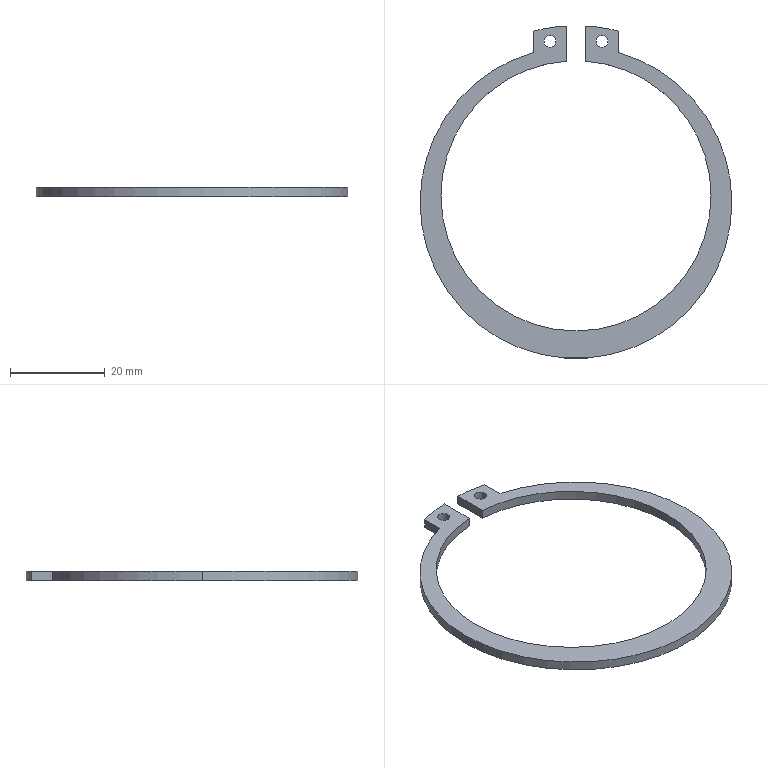Component | SolidWorks | shaft circlip GB894-1 d60-1 | 1 solid | 18 faces | box 65.8 x 70.14 x 2 mm | volume 1778 mm3 | cylinder 12 | plane 6 | commonest cylinder face diameters 2.5 x4 65.8 x3 57 x3 71.8 x2
build123d program:
from build123d import *

# Parameters (mm, degrees)
RING_PROFILE_GB894_1_60_INSTALLED_R = 1.25
RING_BODY_S2_DEPTH                  = 2


with BuildPart() as part:
    # Ring profile GB894.1-60 installed → Ring body s2 (new body)
    with BuildSketch(Plane.XY):
        with BuildLine():
            Line((2, 28.43), (2, 35.844))
            ThreePointArc((2, 35.844), (5.527, 35.472), (9, 34.754))
            Line((9, 34.754), (9, 30.245))
            ThreePointArc((9, 30.245), (0, -34.3), (-9, 30.245))
            Line((-9, 30.245), (-9, 34.754))
            ThreePointArc((-9, 34.754), (-5.527, 35.472), (-2, 35.844))
            Line((-2, 35.844), (-2, 28.43))
            ThreePointArc((-2, 28.43), (0, -28.5), (2, 28.43))
        make_face()
        with Locations((5.5, 32.6)):
            Circle(RING_PROFILE_GB894_1_60_INSTALLED_R, mode=Mode.SUBTRACT)
        with Locations((-5.5, 32.6)):
            Circle(RING_PROFILE_GB894_1_60_INSTALLED_R, mode=Mode.SUBTRACT)
    extrude(amount=RING_BODY_S2_DEPTH)


solid = part.part

# Placed as in the assembly
solid = solid.moved(Location((-85, 178, 139), (0, 0, 0)))
STEP:
#1=CARTESIAN_POINT('',(-3.612,8.291,5.551));
#2=VERTEX_POINT('',#1);
#3=CARTESIAN_POINT('',(-3.514,8.291,5.551));
#4=VERTEX_POINT('',#3);
#5=CARTESIAN_POINT('',(-3.563,8.291,5.551));
#6=DIRECTION('',(0.,0.,1.));
#7=DIRECTION('',(1.,0.,0.));
#8=AXIS2_PLACEMENT_3D('',#5,#6,#7);
#9=CIRCLE('',#8,0.04921);
#10=EDGE_CURVE('',#2,#4,#9,.T.);
#11=ORIENTED_EDGE('',*,*,#10,.T.);
#12=CARTESIAN_POINT('',(-3.514,8.291,5.472));
#13=VERTEX_POINT('',#12);
#14=CARTESIAN_POINT('',(-3.514,8.291,5.551));
#15=DIRECTION('',(0.,0.,-1.));
#16=VECTOR('',#15,39.37);
#17=LINE('',#14,#16);
#18=EDGE_CURVE('',#4,#13,#17,.T.);
#19=ORIENTED_EDGE('',*,*,#18,.T.);
#20=CARTESIAN_POINT('',(-3.612,8.291,5.472));
#21=VERTEX_POINT('',#20);
#22=CARTESIAN_POINT('',(-3.563,8.291,5.472));
#23=DIRECTION('',(0.,0.,1.));
#24=DIRECTION('',(1.,0.,0.));
#25=AXIS2_PLACEMENT_3D('',#22,#23,#24);
#26=CIRCLE('',#25,0.04921);
#27=EDGE_CURVE('',#21,#13,#26,.T.);
#28=ORIENTED_EDGE('',*,*,#27,.F.);
#29=CARTESIAN_POINT('',(-3.612,8.291,5.551));
#30=DIRECTION('',(0.,0.,-1.));
#31=VECTOR('',#30,39.37);
#32=LINE('',#29,#31);
#33=EDGE_CURVE('',#2,#21,#32,.T.);
#34=ORIENTED_EDGE('',*,*,#33,.F.);
#35=EDGE_LOOP('',(#11,#19,#28,#34));
#36=FACE_OUTER_BOUND('',#35,.T.);
#37=CARTESIAN_POINT('',(-3.563,8.291,5.551));
#38=DIRECTION('',(0.,0.,-1.));
#39=DIRECTION('',(-1.,0.,0.));
#40=AXIS2_PLACEMENT_3D('',#37,#38,#39);
#41=CYLINDRICAL_SURFACE('',#40,0.04921);
#42=ADVANCED_FACE('',(#36),#41,.F.);
#43=CARTESIAN_POINT('',(-3.179,8.291,5.551));
#44=VERTEX_POINT('',#43);
#45=CARTESIAN_POINT('',(-3.081,8.291,5.551));
#46=VERTEX_POINT('',#45);
#47=CARTESIAN_POINT('',(-3.13,8.291,5.551));
#48=DIRECTION('',(0.,0.,1.));
#49=DIRECTION('',(1.,0.,0.));
#50=AXIS2_PLACEMENT_3D('',#47,#48,#49);
#51=CIRCLE('',#50,0.04921);
#52=EDGE_CURVE('',#44,#46,#51,.T.);
#53=ORIENTED_EDGE('',*,*,#52,.T.);
#54=CARTESIAN_POINT('',(-3.081,8.291,5.472));
#55=VERTEX_POINT('',#54);
#56=CARTESIAN_POINT('',(-3.081,8.291,5.551));
#57=DIRECTION('',(0.,0.,-1.));
#58=VECTOR('',#57,39.37);
#59=LINE('',#56,#58);
#60=EDGE_CURVE('',#46,#55,#59,.T.);
#61=ORIENTED_EDGE('',*,*,#60,.T.);
#62=CARTESIAN_POINT('',(-3.179,8.291,5.472));
#63=VERTEX_POINT('',#62);
#64=CARTESIAN_POINT('',(-3.13,8.291,5.472));
#65=DIRECTION('',(0.,0.,1.));
#66=DIRECTION('',(1.,0.,0.));
#67=AXIS2_PLACEMENT_3D('',#64,#65,#66);
#68=CIRCLE('',#67,0.04921);
#69=EDGE_CURVE('',#63,#55,#68,.T.);
#70=ORIENTED_EDGE('',*,*,#69,.F.);
#71=CARTESIAN_POINT('',(-3.179,8.291,5.551));
#72=DIRECTION('',(0.,0.,-1.));
#73=VECTOR('',#72,39.37);
#74=LINE('',#71,#73);
#75=EDGE_CURVE('',#44,#63,#74,.T.);
#76=ORIENTED_EDGE('',*,*,#75,.F.);
#77=EDGE_LOOP('',(#53,#61,#70,#76));
#78=FACE_OUTER_BOUND('',#77,.T.);
#79=CARTESIAN_POINT('',(-3.13,8.291,5.551));
#80=DIRECTION('',(0.,0.,-1.));
#81=DIRECTION('',(-1.,0.,0.));
#82=AXIS2_PLACEMENT_3D('',#79,#80,#81);
#83=CYLINDRICAL_SURFACE('',#82,0.04921);
#84=ADVANCED_FACE('',(#78),#83,.F.);
#85=CARTESIAN_POINT('',(-2.051,6.953,5.551));
#86=VERTEX_POINT('',#85);
#87=CARTESIAN_POINT('',(-2.992,8.199,5.551));
#88=VERTEX_POINT('',#87);
#89=CARTESIAN_POINT('',(-3.346,6.953,5.551));
#90=DIRECTION('',(0.,0.,1.));
#91=DIRECTION('',(-1.,0.,0.));
#92=AXIS2_PLACEMENT_3D('',#89,#90,#91);
#93=CIRCLE('',#92,1.295);
#94=EDGE_CURVE('',#86,#88,#93,.T.);
#95=ORIENTED_EDGE('',*,*,#94,.F.);
#96=CARTESIAN_POINT('',(-2.051,6.953,5.472));
#97=VERTEX_POINT('',#96);
#98=CARTESIAN_POINT('',(-2.051,6.953,5.551));
#99=DIRECTION('',(0.,0.,-1.));
#100=VECTOR('',#99,39.37);
#101=LINE('',#98,#100);
#102=EDGE_CURVE('',#86,#97,#101,.T.);
#103=ORIENTED_EDGE('',*,*,#102,.T.);
#104=CARTESIAN_POINT('',(-2.992,8.199,5.472));
#105=VERTEX_POINT('',#104);
#106=CARTESIAN_POINT('',(-3.346,6.953,5.472));
#107=DIRECTION('',(0.,0.,1.));
#108=DIRECTION('',(-1.,0.,0.));
#109=AXIS2_PLACEMENT_3D('',#106,#107,#108);
#110=CIRCLE('',#109,1.295);
#111=EDGE_CURVE('',#97,#105,#110,.T.);
#112=ORIENTED_EDGE('',*,*,#111,.T.);
#113=CARTESIAN_POINT('',(-2.992,8.199,5.551));
#114=DIRECTION('',(0.,0.,-1.));
#115=VECTOR('',#114,39.37);
#116=LINE('',#113,#115);
#117=EDGE_CURVE('',#88,#105,#116,.T.);
#118=ORIENTED_EDGE('',*,*,#117,.F.);
#119=EDGE_LOOP('',(#95,#103,#112,#118));
#120=FACE_OUTER_BOUND('',#119,.T.);
#121=CARTESIAN_POINT('',(-3.346,6.953,5.551));
#122=DIRECTION('',(0.,0.,-1.));
#123=DIRECTION('',(-1.,0.,0.));
#124=AXIS2_PLACEMENT_3D('',#121,#122,#123);
#125=CYLINDRICAL_SURFACE('',#124,1.295);
#126=ADVANCED_FACE('',(#120),#125,.T.);
#127=ORIENTED_EDGE('',*,*,#102,.F.);
#128=CARTESIAN_POINT('',(-4.642,6.953,5.551));
#129=VERTEX_POINT('',#128);
#130=CARTESIAN_POINT('',(-3.346,6.953,5.551));
#131=DIRECTION('',(0.,0.,1.));
#132=DIRECTION('',(-1.,0.,0.));
#133=AXIS2_PLACEMENT_3D('',#130,#131,#132);
#134=CIRCLE('',#133,1.295);
#135=EDGE_CURVE('',#129,#86,#134,.T.);
#136=ORIENTED_EDGE('',*,*,#135,.F.);
#137=CARTESIAN_POINT('',(-4.642,6.953,5.472));
#138=VERTEX_POINT('',#137);
#139=CARTESIAN_POINT('',(-4.642,6.953,5.551));
#140=DIRECTION('',(0.,0.,-1.));
#141=VECTOR('',#140,39.37);
#142=LINE('',#139,#141);
#143=EDGE_CURVE('',#129,#138,#142,.T.);
#144=ORIENTED_EDGE('',*,*,#143,.T.);
#145=CARTESIAN_POINT('',(-3.346,6.953,5.472));
#146=DIRECTION('',(0.,0.,1.));
#147=DIRECTION('',(-1.,0.,0.));
#148=AXIS2_PLACEMENT_3D('',#145,#146,#147);
#149=CIRCLE('',#148,1.295);
#150=EDGE_CURVE('',#138,#97,#149,.T.);
#151=ORIENTED_EDGE('',*,*,#150,.T.);
#152=EDGE_LOOP('',(#127,#136,#144,#151));
#153=FACE_OUTER_BOUND('',#152,.T.);
#154=CARTESIAN_POINT('',(-3.346,6.953,5.551));
#155=DIRECTION('',(0.,0.,-1.));
#156=DIRECTION('',(-1.,0.,0.));
#157=AXIS2_PLACEMENT_3D('',#154,#155,#156);
#158=CYLINDRICAL_SURFACE('',#157,1.295);
#159=ADVANCED_FACE('',(#153),#158,.T.);
#160=CARTESIAN_POINT('',(-2.224,7.008,5.551));
#161=VERTEX_POINT('',#160);
#162=CARTESIAN_POINT('',(-4.469,7.008,5.551));
#163=VERTEX_POINT('',#162);
#164=CARTESIAN_POINT('',(-3.346,7.008,5.551));
#165=DIRECTION('',(0.,0.,-1.));
#166=DIRECTION('',(1.,0.,0.));
#167=AXIS2_PLACEMENT_3D('',#164,#165,#166);
#168=CIRCLE('',#167,1.122);
#169=EDGE_CURVE('',#161,#163,#168,.T.);
#170=ORIENTED_EDGE('',*,*,#169,.F.);
#171=CARTESIAN_POINT('',(-2.224,7.008,5.472));
#172=VERTEX_POINT('',#171);
#173=CARTESIAN_POINT('',(-2.224,7.008,5.551));
#174=DIRECTION('',(0.,0.,-1.));
#175=VECTOR('',#174,39.37);
#176=LINE('',#173,#175);
#177=EDGE_CURVE('',#161,#172,#176,.T.);
#178=ORIENTED_EDGE('',*,*,#177,.T.);
#179=CARTESIAN_POINT('',(-4.469,7.008,5.472));
#180=VERTEX_POINT('',#179);
#181=CARTESIAN_POINT('',(-3.346,7.008,5.472));
#182=DIRECTION('',(0.,0.,-1.));
#183=DIRECTION('',(1.,0.,0.));
#184=AXIS2_PLACEMENT_3D('',#181,#182,#183);
#185=CIRCLE('',#184,1.122);
#186=EDGE_CURVE('',#172,#180,#185,.T.);
#187=ORIENTED_EDGE('',*,*,#186,.T.);
#188=CARTESIAN_POINT('',(-4.469,7.008,5.551));
#189=DIRECTION('',(0.,0.,-1.));
#190=VECTOR('',#189,39.37);
#191=LINE('',#188,#190);
#192=EDGE_CURVE('',#163,#180,#191,.T.);
#193=ORIENTED_EDGE('',*,*,#192,.F.);
#194=EDGE_LOOP('',(#170,#178,#187,#193));
#195=FACE_OUTER_BOUND('',#194,.T.);
#196=CARTESIAN_POINT('',(-3.346,7.008,5.551));
#197=DIRECTION('',(0.,0.,-1.));
#198=DIRECTION('',(-1.,0.,0.));
#199=AXIS2_PLACEMENT_3D('',#196,#197,#198);
#200=CYLINDRICAL_SURFACE('',#199,1.122);
#201=ADVANCED_FACE('',(#195),#200,.F.);
#202=CARTESIAN_POINT('',(-3.425,8.127,5.551));
#203=VERTEX_POINT('',#202);
#204=CARTESIAN_POINT('',(-3.346,7.008,5.551));
#205=DIRECTION('',(0.,0.,-1.));
#206=DIRECTION('',(1.,0.,0.));
#207=AXIS2_PLACEMENT_3D('',#204,#205,#206);
#208=CIRCLE('',#207,1.122);
#209=EDGE_CURVE('',#163,#203,#208,.T.);
#210=ORIENTED_EDGE('',*,*,#209,.F.);
#211=ORIENTED_EDGE('',*,*,#192,.T.);
#212=CARTESIAN_POINT('',(-3.425,8.127,5.472));
#213=VERTEX_POINT('',#212);
#214=CARTESIAN_POINT('',(-3.346,7.008,5.472));
#215=DIRECTION('',(0.,0.,-1.));
#216=DIRECTION('',(1.,0.,0.));
#217=AXIS2_PLACEMENT_3D('',#214,#215,#216);
#218=CIRCLE('',#217,1.122);
#219=EDGE_CURVE('',#180,#213,#218,.T.);
#220=ORIENTED_EDGE('',*,*,#219,.T.);
#221=CARTESIAN_POINT('',(-3.425,8.127,5.551));
#222=DIRECTION('',(0.,0.,-1.));
#223=VECTOR('',#222,39.37);
#224=LINE('',#221,#223);
#225=EDGE_CURVE('',#203,#213,#224,.T.);
#226=ORIENTED_EDGE('',*,*,#225,.F.);
#227=EDGE_LOOP('',(#210,#211,#220,#226));
#228=FACE_OUTER_BOUND('',#227,.T.);
#229=CARTESIAN_POINT('',(-3.346,7.008,5.551));
#230=DIRECTION('',(0.,0.,-1.));
#231=DIRECTION('',(-1.,0.,0.));
#232=AXIS2_PLACEMENT_3D('',#229,#230,#231);
#233=CYLINDRICAL_SURFACE('',#232,1.122);
#234=ADVANCED_FACE('',(#228),#233,.F.);
#235=ORIENTED_EDGE('',*,*,#52,.F.);
#236=CARTESIAN_POINT('',(-3.13,8.291,5.551));
#237=DIRECTION('',(0.,0.,1.));
#238=DIRECTION('',(1.,0.,0.));
#239=AXIS2_PLACEMENT_3D('',#236,#237,#238);
#240=CIRCLE('',#239,0.04921);
#241=EDGE_CURVE('',#46,#44,#240,.T.);
#242=ORIENTED_EDGE('',*,*,#241,.F.);
#243=EDGE_LOOP('',(#235,#242));
#244=FACE_BOUND('',#243,.T.);
#245=CARTESIAN_POINT('',(-3.268,8.127,5.551));
#246=VERTEX_POINT('',#245);
#247=CARTESIAN_POINT('',(-3.346,7.008,5.551));
#248=DIRECTION('',(0.,0.,-1.));
#249=DIRECTION('',(1.,0.,0.));
#250=AXIS2_PLACEMENT_3D('',#247,#248,#249);
#251=CIRCLE('',#250,1.122);
#252=EDGE_CURVE('',#246,#161,#251,.T.);
#253=ORIENTED_EDGE('',*,*,#252,.T.);
#254=ORIENTED_EDGE('',*,*,#169,.T.);
#255=ORIENTED_EDGE('',*,*,#209,.T.);
#256=CARTESIAN_POINT('',(-3.425,8.419,5.551));
#257=VERTEX_POINT('',#256);
#258=CARTESIAN_POINT('',(-3.425,8.419,5.551));
#259=DIRECTION('',(0.,1.,0.));
#260=VECTOR('',#259,39.37);
#261=LINE('',#258,#260);
#262=EDGE_CURVE('',#203,#257,#261,.T.);
#263=ORIENTED_EDGE('',*,*,#262,.T.);
#264=CARTESIAN_POINT('',(-3.701,8.376,5.551));
#265=VERTEX_POINT('',#264);
#266=CARTESIAN_POINT('',(-3.346,7.008,5.551));
#267=DIRECTION('',(0.,0.,1.));
#268=DIRECTION('',(-1.,0.,0.));
#269=AXIS2_PLACEMENT_3D('',#266,#267,#268);
#270=CIRCLE('',#269,1.413);
#271=EDGE_CURVE('',#257,#265,#270,.T.);
#272=ORIENTED_EDGE('',*,*,#271,.T.);
#273=CARTESIAN_POINT('',(-3.701,8.199,5.551));
#274=VERTEX_POINT('',#273);
#275=CARTESIAN_POINT('',(-3.701,8.199,5.551));
#276=DIRECTION('',(0.,-1.,0.));
#277=VECTOR('',#276,39.37);
#278=LINE('',#275,#277);
#279=EDGE_CURVE('',#265,#274,#278,.T.);
#280=ORIENTED_EDGE('',*,*,#279,.T.);
#281=CARTESIAN_POINT('',(-3.346,6.953,5.551));
#282=DIRECTION('',(0.,0.,1.));
#283=DIRECTION('',(-1.,0.,0.));
#284=AXIS2_PLACEMENT_3D('',#281,#282,#283);
#285=CIRCLE('',#284,1.295);
#286=EDGE_CURVE('',#274,#129,#285,.T.);
#287=ORIENTED_EDGE('',*,*,#286,.T.);
#288=ORIENTED_EDGE('',*,*,#135,.T.);
#289=ORIENTED_EDGE('',*,*,#94,.T.);
#290=CARTESIAN_POINT('',(-2.992,8.376,5.551));
#291=VERTEX_POINT('',#290);
#292=CARTESIAN_POINT('',(-2.992,8.376,5.551));
#293=DIRECTION('',(0.,1.,0.));
#294=VECTOR('',#293,39.37);
#295=LINE('',#292,#294);
#296=EDGE_CURVE('',#88,#291,#295,.T.);
#297=ORIENTED_EDGE('',*,*,#296,.T.);
#298=CARTESIAN_POINT('',(-3.268,8.419,5.551));
#299=VERTEX_POINT('',#298);
#300=CARTESIAN_POINT('',(-3.346,7.008,5.551));
#301=DIRECTION('',(0.,0.,1.));
#302=DIRECTION('',(-1.,0.,0.));
#303=AXIS2_PLACEMENT_3D('',#300,#301,#302);
#304=CIRCLE('',#303,1.413);
#305=EDGE_CURVE('',#291,#299,#304,.T.);
#306=ORIENTED_EDGE('',*,*,#305,.T.);
#307=CARTESIAN_POINT('',(-3.268,8.127,5.551));
#308=DIRECTION('',(0.,-1.,0.));
#309=VECTOR('',#308,39.37);
#310=LINE('',#307,#309);
#311=EDGE_CURVE('',#299,#246,#310,.T.);
#312=ORIENTED_EDGE('',*,*,#311,.T.);
#313=EDGE_LOOP('',(#253,#254,#255,#263,#272,#280,#287,#288,#289,#297,#306,#312));
#314=FACE_OUTER_BOUND('',#313,.T.);
#315=ORIENTED_EDGE('',*,*,#10,.F.);
#316=CARTESIAN_POINT('',(-3.563,8.291,5.551));
#317=DIRECTION('',(0.,0.,1.));
#318=DIRECTION('',(1.,0.,0.));
#319=AXIS2_PLACEMENT_3D('',#316,#317,#318);
#320=CIRCLE('',#319,0.04921);
#321=EDGE_CURVE('',#4,#2,#320,.T.);
#322=ORIENTED_EDGE('',*,*,#321,.F.);
#323=EDGE_LOOP('',(#315,#322));
#324=FACE_BOUND('',#323,.T.);
#325=CARTESIAN_POINT('',(-3.346,7.008,5.551));
#326=DIRECTION('',(0.,0.,1.));
#327=DIRECTION('',(1.,0.,0.));
#328=AXIS2_PLACEMENT_3D('',#325,#326,#327);
#329=PLANE('',#328);
#330=ADVANCED_FACE('',(#244,#314,#324),#329,.T.);
#331=CARTESIAN_POINT('',(-3.268,8.127,5.472));
#332=VERTEX_POINT('',#331);
#333=CARTESIAN_POINT('',(-3.346,7.008,5.472));
#334=DIRECTION('',(0.,0.,-1.));
#335=DIRECTION('',(1.,0.,0.));
#336=AXIS2_PLACEMENT_3D('',#333,#334,#335);
#337=CIRCLE('',#336,1.122);
#338=EDGE_CURVE('',#332,#172,#337,.T.);
#339=ORIENTED_EDGE('',*,*,#338,.F.);
#340=CARTESIAN_POINT('',(-3.268,8.419,5.472));
#341=VERTEX_POINT('',#340);
#342=CARTESIAN_POINT('',(-3.268,8.127,5.472));
#343=DIRECTION('',(0.,-1.,0.));
#344=VECTOR('',#343,39.37);
#345=LINE('',#342,#344);
#346=EDGE_CURVE('',#341,#332,#345,.T.);
#347=ORIENTED_EDGE('',*,*,#346,.F.);
#348=CARTESIAN_POINT('',(-2.992,8.376,5.472));
#349=VERTEX_POINT('',#348);
#350=CARTESIAN_POINT('',(-3.346,7.008,5.472));
#351=DIRECTION('',(0.,0.,1.));
#352=DIRECTION('',(-1.,0.,0.));
#353=AXIS2_PLACEMENT_3D('',#350,#351,#352);
#354=CIRCLE('',#353,1.413);
#355=EDGE_CURVE('',#349,#341,#354,.T.);
#356=ORIENTED_EDGE('',*,*,#355,.F.);
#357=CARTESIAN_POINT('',(-2.992,8.376,5.472));
#358=DIRECTION('',(0.,1.,0.));
#359=VECTOR('',#358,39.37);
#360=LINE('',#357,#359);
#361=EDGE_CURVE('',#105,#349,#360,.T.);
#362=ORIENTED_EDGE('',*,*,#361,.F.);
#363=ORIENTED_EDGE('',*,*,#111,.F.);
#364=ORIENTED_EDGE('',*,*,#150,.F.);
#365=CARTESIAN_POINT('',(-3.701,8.199,5.472));
#366=VERTEX_POINT('',#365);
#367=CARTESIAN_POINT('',(-3.346,6.953,5.472));
#368=DIRECTION('',(0.,0.,1.));
#369=DIRECTION('',(-1.,0.,0.));
#370=AXIS2_PLACEMENT_3D('',#367,#368,#369);
#371=CIRCLE('',#370,1.295);
#372=EDGE_CURVE('',#366,#138,#371,.T.);
#373=ORIENTED_EDGE('',*,*,#372,.F.);
#374=CARTESIAN_POINT('',(-3.701,8.376,5.472));
#375=VERTEX_POINT('',#374);
#376=CARTESIAN_POINT('',(-3.701,8.199,5.472));
#377=DIRECTION('',(0.,-1.,0.));
#378=VECTOR('',#377,39.37);
#379=LINE('',#376,#378);
#380=EDGE_CURVE('',#375,#366,#379,.T.);
#381=ORIENTED_EDGE('',*,*,#380,.F.);
#382=CARTESIAN_POINT('',(-3.425,8.419,5.472));
#383=VERTEX_POINT('',#382);
#384=CARTESIAN_POINT('',(-3.346,7.008,5.472));
#385=DIRECTION('',(0.,0.,1.));
#386=DIRECTION('',(-1.,0.,0.));
#387=AXIS2_PLACEMENT_3D('',#384,#385,#386);
#388=CIRCLE('',#387,1.413);
#389=EDGE_CURVE('',#383,#375,#388,.T.);
#390=ORIENTED_EDGE('',*,*,#389,.F.);
#391=CARTESIAN_POINT('',(-3.425,8.419,5.472));
#392=DIRECTION('',(0.,1.,0.));
#393=VECTOR('',#392,39.37);
#394=LINE('',#391,#393);
#395=EDGE_CURVE('',#213,#383,#394,.T.);
#396=ORIENTED_EDGE('',*,*,#395,.F.);
#397=ORIENTED_EDGE('',*,*,#219,.F.);
#398=ORIENTED_EDGE('',*,*,#186,.F.);
#399=EDGE_LOOP('',(#339,#347,#356,#362,#363,#364,#373,#381,#390,#396,#397,#398));
#400=FACE_OUTER_BOUND('',#399,.T.);
#401=ORIENTED_EDGE('',*,*,#69,.T.);
#402=CARTESIAN_POINT('',(-3.13,8.291,5.472));
#403=DIRECTION('',(0.,0.,1.));
#404=DIRECTION('',(1.,0.,0.));
#405=AXIS2_PLACEMENT_3D('',#402,#403,#404);
#406=CIRCLE('',#405,0.04921);
#407=EDGE_CURVE('',#55,#63,#406,.T.);
#408=ORIENTED_EDGE('',*,*,#407,.T.);
#409=EDGE_LOOP('',(#401,#408));
#410=FACE_BOUND('',#409,.T.);
#411=ORIENTED_EDGE('',*,*,#27,.T.);
#412=CARTESIAN_POINT('',(-3.563,8.291,5.472));
#413=DIRECTION('',(0.,0.,1.));
#414=DIRECTION('',(1.,0.,0.));
#415=AXIS2_PLACEMENT_3D('',#412,#413,#414);
#416=CIRCLE('',#415,0.04921);
#417=EDGE_CURVE('',#13,#21,#416,.T.);
#418=ORIENTED_EDGE('',*,*,#417,.T.);
#419=EDGE_LOOP('',(#411,#418));
#420=FACE_BOUND('',#419,.T.);
#421=CARTESIAN_POINT('',(-3.346,7.008,5.472));
#422=DIRECTION('',(0.,0.,1.));
#423=DIRECTION('',(1.,0.,0.));
#424=AXIS2_PLACEMENT_3D('',#421,#422,#423);
#425=PLANE('',#424);
#426=ADVANCED_FACE('',(#400,#410,#420),#425,.F.);
#427=ORIENTED_EDGE('',*,*,#177,.F.);
#428=ORIENTED_EDGE('',*,*,#252,.F.);
#429=CARTESIAN_POINT('',(-3.268,8.127,5.551));
#430=DIRECTION('',(0.,0.,-1.));
#431=VECTOR('',#430,39.37);
#432=LINE('',#429,#431);
#433=EDGE_CURVE('',#246,#332,#432,.T.);
#434=ORIENTED_EDGE('',*,*,#433,.T.);
#435=ORIENTED_EDGE('',*,*,#338,.T.);
#436=EDGE_LOOP('',(#427,#428,#434,#435));
#437=FACE_OUTER_BOUND('',#436,.T.);
#438=CARTESIAN_POINT('',(-3.346,7.008,5.551));
#439=DIRECTION('',(0.,0.,-1.));
#440=DIRECTION('',(-1.,0.,0.));
#441=AXIS2_PLACEMENT_3D('',#438,#439,#440);
#442=CYLINDRICAL_SURFACE('',#441,1.122);
#443=ADVANCED_FACE('',(#437),#442,.F.);
#444=ORIENTED_EDGE('',*,*,#395,.T.);
#445=CARTESIAN_POINT('',(-3.425,8.419,5.551));
#446=DIRECTION('',(0.,0.,-1.));
#447=VECTOR('',#446,39.37);
#448=LINE('',#445,#447);
#449=EDGE_CURVE('',#257,#383,#448,.T.);
#450=ORIENTED_EDGE('',*,*,#449,.F.);
#451=ORIENTED_EDGE('',*,*,#262,.F.);
#452=ORIENTED_EDGE('',*,*,#225,.T.);
#453=EDGE_LOOP('',(#444,#450,#451,#452));
#454=FACE_OUTER_BOUND('',#453,.T.);
#455=CARTESIAN_POINT('',(-3.425,8.419,5.551));
#456=DIRECTION('',(-1.,0.,0.));
#457=DIRECTION('',(0.,0.,1.));
#458=AXIS2_PLACEMENT_3D('',#455,#456,#457);
#459=PLANE('',#458);
#460=ADVANCED_FACE('',(#454),#459,.F.);
#461=ORIENTED_EDGE('',*,*,#389,.T.);
#462=CARTESIAN_POINT('',(-3.701,8.376,5.551));
#463=DIRECTION('',(0.,0.,-1.));
#464=VECTOR('',#463,39.37);
#465=LINE('',#462,#464);
#466=EDGE_CURVE('',#265,#375,#465,.T.);
#467=ORIENTED_EDGE('',*,*,#466,.F.);
#468=ORIENTED_EDGE('',*,*,#271,.F.);
#469=ORIENTED_EDGE('',*,*,#449,.T.);
#470=EDGE_LOOP('',(#461,#467,#468,#469));
#471=FACE_OUTER_BOUND('',#470,.T.);
#472=CARTESIAN_POINT('',(-3.346,7.008,5.551));
#473=DIRECTION('',(0.,0.,-1.));
#474=DIRECTION('',(-1.,0.,0.));
#475=AXIS2_PLACEMENT_3D('',#472,#473,#474);
#476=CYLINDRICAL_SURFACE('',#475,1.413);
#477=ADVANCED_FACE('',(#471),#476,.T.);
#478=ORIENTED_EDGE('',*,*,#380,.T.);
#479=CARTESIAN_POINT('',(-3.701,8.199,5.551));
#480=DIRECTION('',(0.,0.,-1.));
#481=VECTOR('',#480,39.37);
#482=LINE('',#479,#481);
#483=EDGE_CURVE('',#274,#366,#482,.T.);
#484=ORIENTED_EDGE('',*,*,#483,.F.);
#485=ORIENTED_EDGE('',*,*,#279,.F.);
#486=ORIENTED_EDGE('',*,*,#466,.T.);
#487=EDGE_LOOP('',(#478,#484,#485,#486));
#488=FACE_OUTER_BOUND('',#487,.T.);
#489=CARTESIAN_POINT('',(-3.701,8.199,5.551));
#490=DIRECTION('',(1.,0.,0.));
#491=DIRECTION('',(0.,0.,-1.));
#492=AXIS2_PLACEMENT_3D('',#489,#490,#491);
#493=PLANE('',#492);
#494=ADVANCED_FACE('',(#488),#493,.F.);
#495=ORIENTED_EDGE('',*,*,#143,.F.);
#496=ORIENTED_EDGE('',*,*,#286,.F.);
#497=ORIENTED_EDGE('',*,*,#483,.T.);
#498=ORIENTED_EDGE('',*,*,#372,.T.);
#499=EDGE_LOOP('',(#495,#496,#497,#498));
#500=FACE_OUTER_BOUND('',#499,.T.);
#501=CARTESIAN_POINT('',(-3.346,6.953,5.551));
#502=DIRECTION('',(0.,0.,-1.));
#503=DIRECTION('',(-1.,0.,0.));
#504=AXIS2_PLACEMENT_3D('',#501,#502,#503);
#505=CYLINDRICAL_SURFACE('',#504,1.295);
#506=ADVANCED_FACE('',(#500),#505,.T.);
#507=ORIENTED_EDGE('',*,*,#361,.T.);
#508=CARTESIAN_POINT('',(-2.992,8.376,5.551));
#509=DIRECTION('',(0.,0.,-1.));
#510=VECTOR('',#509,39.37);
#511=LINE('',#508,#510);
#512=EDGE_CURVE('',#291,#349,#511,.T.);
#513=ORIENTED_EDGE('',*,*,#512,.F.);
#514=ORIENTED_EDGE('',*,*,#296,.F.);
#515=ORIENTED_EDGE('',*,*,#117,.T.);
#516=EDGE_LOOP('',(#507,#513,#514,#515));
#517=FACE_OUTER_BOUND('',#516,.T.);
#518=CARTESIAN_POINT('',(-2.992,8.376,5.551));
#519=DIRECTION('',(-1.,0.,0.));
#520=DIRECTION('',(0.,0.,1.));
#521=AXIS2_PLACEMENT_3D('',#518,#519,#520);
#522=PLANE('',#521);
#523=ADVANCED_FACE('',(#517),#522,.F.);
#524=ORIENTED_EDGE('',*,*,#355,.T.);
#525=CARTESIAN_POINT('',(-3.268,8.419,5.551));
#526=DIRECTION('',(0.,0.,-1.));
#527=VECTOR('',#526,39.37);
#528=LINE('',#525,#527);
#529=EDGE_CURVE('',#299,#341,#528,.T.);
#530=ORIENTED_EDGE('',*,*,#529,.F.);
#531=ORIENTED_EDGE('',*,*,#305,.F.);
#532=ORIENTED_EDGE('',*,*,#512,.T.);
#533=EDGE_LOOP('',(#524,#530,#531,#532));
#534=FACE_OUTER_BOUND('',#533,.T.);
#535=CARTESIAN_POINT('',(-3.346,7.008,5.551));
#536=DIRECTION('',(0.,0.,-1.));
#537=DIRECTION('',(-1.,0.,0.));
#538=AXIS2_PLACEMENT_3D('',#535,#536,#537);
#539=CYLINDRICAL_SURFACE('',#538,1.413);
#540=ADVANCED_FACE('',(#534),#539,.T.);
#541=ORIENTED_EDGE('',*,*,#346,.T.);
#542=ORIENTED_EDGE('',*,*,#433,.F.);
#543=ORIENTED_EDGE('',*,*,#311,.F.);
#544=ORIENTED_EDGE('',*,*,#529,.T.);
#545=EDGE_LOOP('',(#541,#542,#543,#544));
#546=FACE_OUTER_BOUND('',#545,.T.);
#547=CARTESIAN_POINT('',(-3.268,8.127,5.551));
#548=DIRECTION('',(1.,0.,0.));
#549=DIRECTION('',(0.,0.,-1.));
#550=AXIS2_PLACEMENT_3D('',#547,#548,#549);
#551=PLANE('',#550);
#552=ADVANCED_FACE('',(#546),#551,.F.);
#553=ORIENTED_EDGE('',*,*,#60,.F.);
#554=ORIENTED_EDGE('',*,*,#241,.T.);
#555=ORIENTED_EDGE('',*,*,#75,.T.);
#556=ORIENTED_EDGE('',*,*,#407,.F.);
#557=EDGE_LOOP('',(#553,#554,#555,#556));
#558=FACE_OUTER_BOUND('',#557,.T.);
#559=CARTESIAN_POINT('',(-3.13,8.291,5.551));
#560=DIRECTION('',(0.,0.,-1.));
#561=DIRECTION('',(-1.,0.,0.));
#562=AXIS2_PLACEMENT_3D('',#559,#560,#561);
#563=CYLINDRICAL_SURFACE('',#562,0.04921);
#564=ADVANCED_FACE('',(#558),#563,.F.);
#565=ORIENTED_EDGE('',*,*,#18,.F.);
#566=ORIENTED_EDGE('',*,*,#321,.T.);
#567=ORIENTED_EDGE('',*,*,#33,.T.);
#568=ORIENTED_EDGE('',*,*,#417,.F.);
#569=EDGE_LOOP('',(#565,#566,#567,#568));
#570=FACE_OUTER_BOUND('',#569,.T.);
#571=CARTESIAN_POINT('',(-3.563,8.291,5.551));
#572=DIRECTION('',(0.,0.,-1.));
#573=DIRECTION('',(-1.,0.,0.));
#574=AXIS2_PLACEMENT_3D('',#571,#572,#573);
#575=CYLINDRICAL_SURFACE('',#574,0.04921);
#576=ADVANCED_FACE('',(#570),#575,.F.);
#577=CLOSED_SHELL('',(#42,#84,#126,#159,#201,#234,#330,#426,#443,#460,#477,#494,#506,#523,#540,#552,#564,#576));
#578=MANIFOLD_SOLID_BREP('',#577);
#579=CARTESIAN_POINT('',(0.,0.,0.));
#580=DIRECTION('',(0.,0.,1.));
#581=DIRECTION('',(1.,0.,0.));
#582=AXIS2_PLACEMENT_3D('',#579,#580,#581);
#583=(LENGTH_UNIT()NAMED_UNIT(*)SI_UNIT($,.METRE.));
#584=LENGTH_MEASURE_WITH_UNIT(LENGTH_MEASURE(0.0254),#583);
#585=DIMENSIONAL_EXPONENTS(1.,0.,0.,0.,0.,0.,0.);
#586=(CONVERSION_BASED_UNIT('',#584)LENGTH_UNIT()NAMED_UNIT(#585));
#587=UNCERTAINTY_MEASURE_WITH_UNIT(LENGTH_MEASURE(0.00001),#586,'','');
#588=(NAMED_UNIT(*)PLANE_ANGLE_UNIT()SI_UNIT($,.RADIAN.));
#589=(NAMED_UNIT(*)SI_UNIT($,.STERADIAN.)SOLID_ANGLE_UNIT());
#590=(GEOMETRIC_REPRESENTATION_CONTEXT(3)GLOBAL_UNCERTAINTY_ASSIGNED_CONTEXT((#587))GLOBAL_UNIT_ASSIGNED_CONTEXT((#586,#588,#589))REPRESENTATION_CONTEXT('',''));
#591=ADVANCED_BREP_SHAPE_REPRESENTATION('',(#578,#582),#590);
#592=COLOUR_RGB('',0.7922,0.8196,0.9333);
#593=FILL_AREA_STYLE_COLOUR('',#592);
#594=FILL_AREA_STYLE('',(#593));
#595=SURFACE_STYLE_FILL_AREA(#594);
#596=SURFACE_SIDE_STYLE('',(#595));
#597=SURFACE_STYLE_USAGE(.BOTH.,#596);
#598=PRESENTATION_STYLE_ASSIGNMENT((#597));
#599=STYLED_ITEM('',(#598),#578);
#600=PRESENTATION_LAYER_ASSIGNMENT('','',(#599));
#601=(LENGTH_UNIT()NAMED_UNIT(*)SI_UNIT($,.METRE.));
#602=LENGTH_MEASURE_WITH_UNIT(LENGTH_MEASURE(0.0254),#601);
#603=DIMENSIONAL_EXPONENTS(1.,0.,0.,0.,0.,0.,0.);
#604=(CONVERSION_BASED_UNIT('',#602)LENGTH_UNIT()NAMED_UNIT(#603));
#605=UNCERTAINTY_MEASURE_WITH_UNIT(LENGTH_MEASURE(0.00001),#604,'','');
#606=(NAMED_UNIT(*)PLANE_ANGLE_UNIT()SI_UNIT($,.RADIAN.));
#607=(NAMED_UNIT(*)SI_UNIT($,.STERADIAN.)SOLID_ANGLE_UNIT());
#608=(GEOMETRIC_REPRESENTATION_CONTEXT(3)GLOBAL_UNCERTAINTY_ASSIGNED_CONTEXT((#605))GLOBAL_UNIT_ASSIGNED_CONTEXT((#604,#606,#607))REPRESENTATION_CONTEXT('',''));
#609=MECHANICAL_DESIGN_GEOMETRIC_PRESENTATION_REPRESENTATION('',(#599),#608);